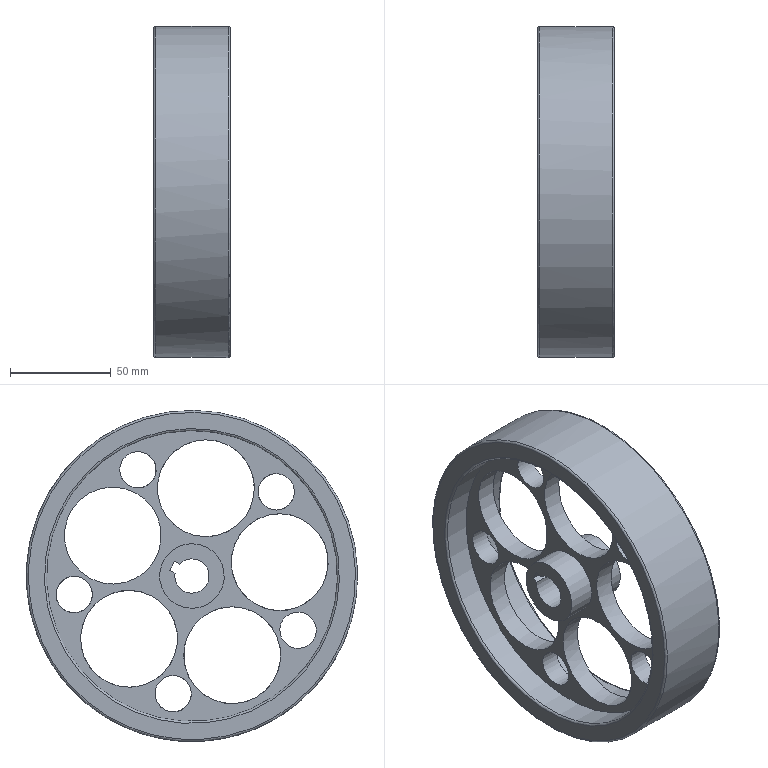Component | NX | FLYWHEEL | 1 solid | 29 faces | volume 254228 mm3 | cylinder 16 | plane 9 | torus 4 | commonest cylinder face diameters 18 x5 48 x5 144 x2 32 x2 164 x1 17 x1